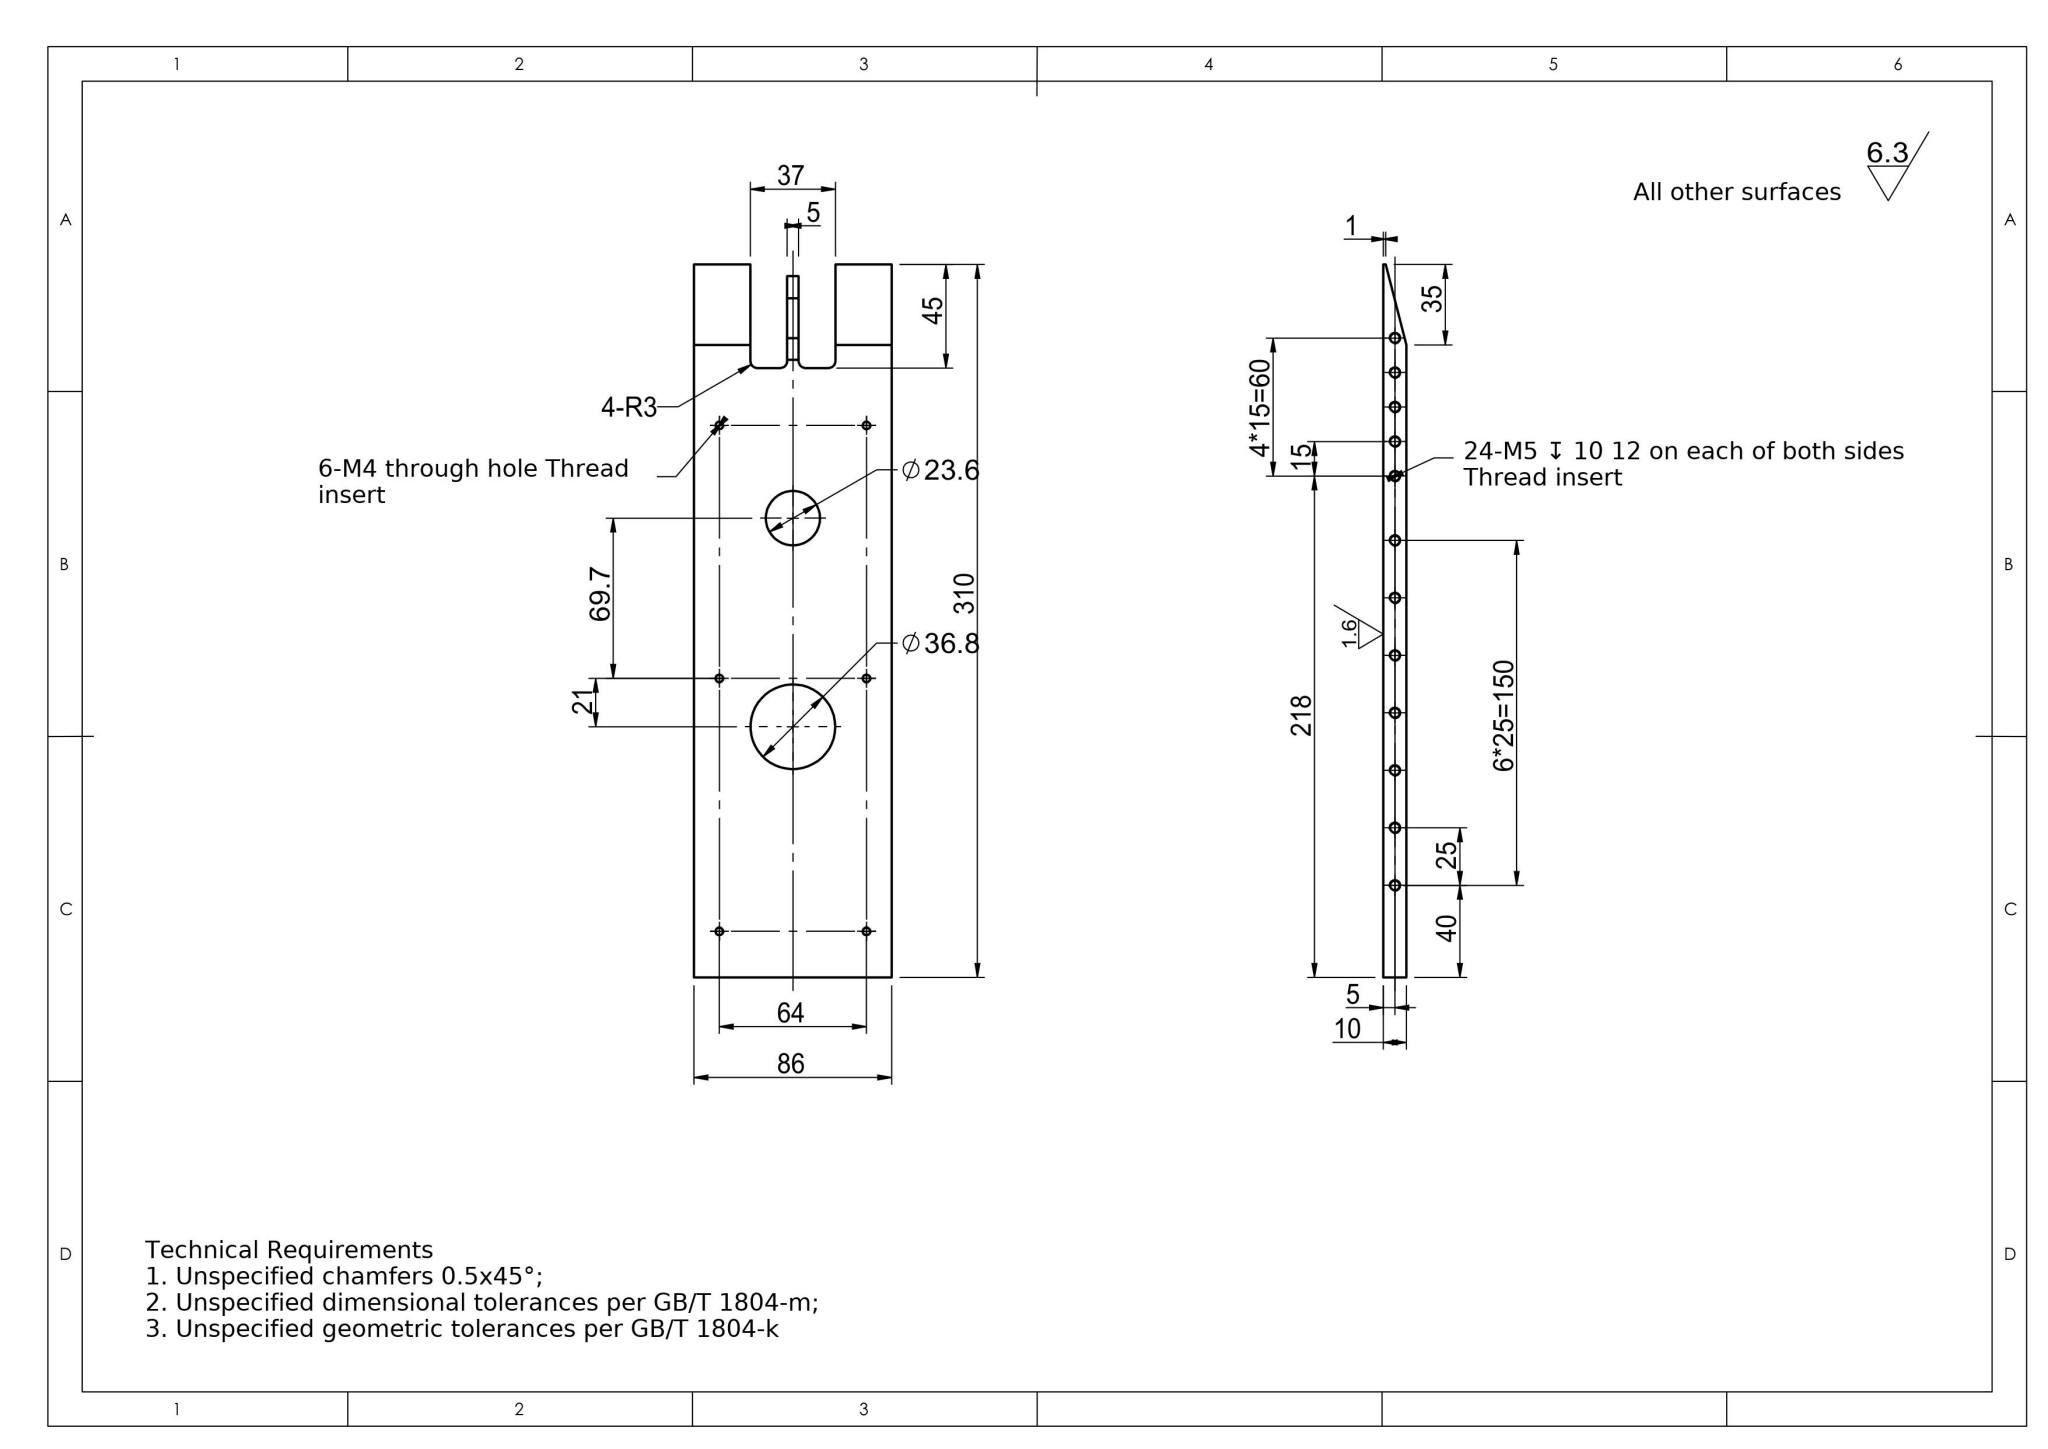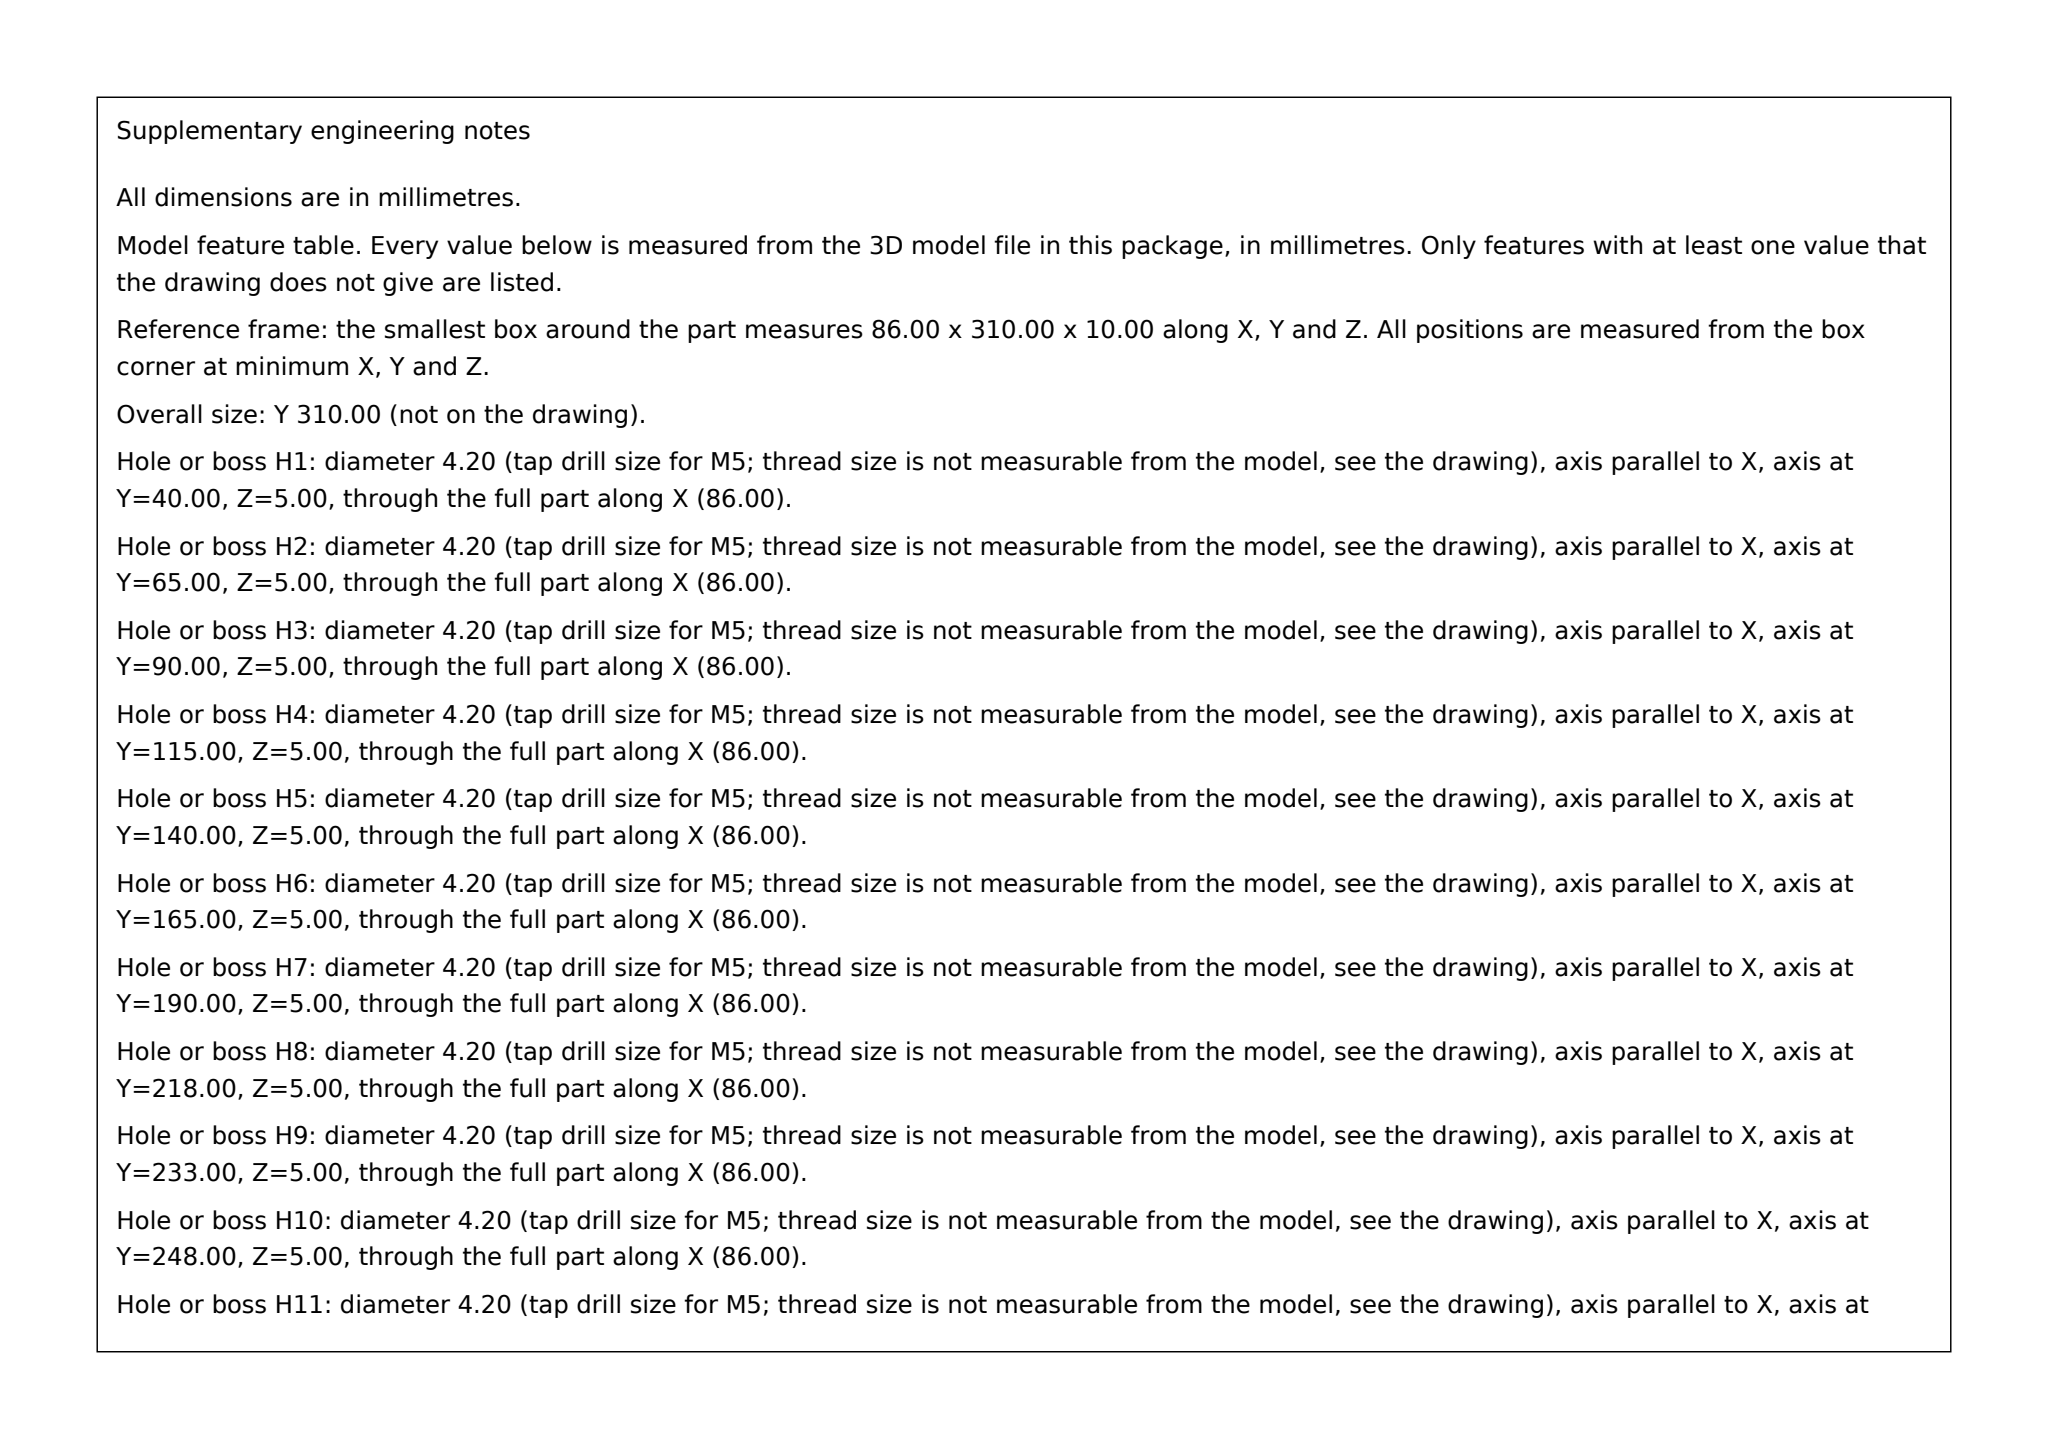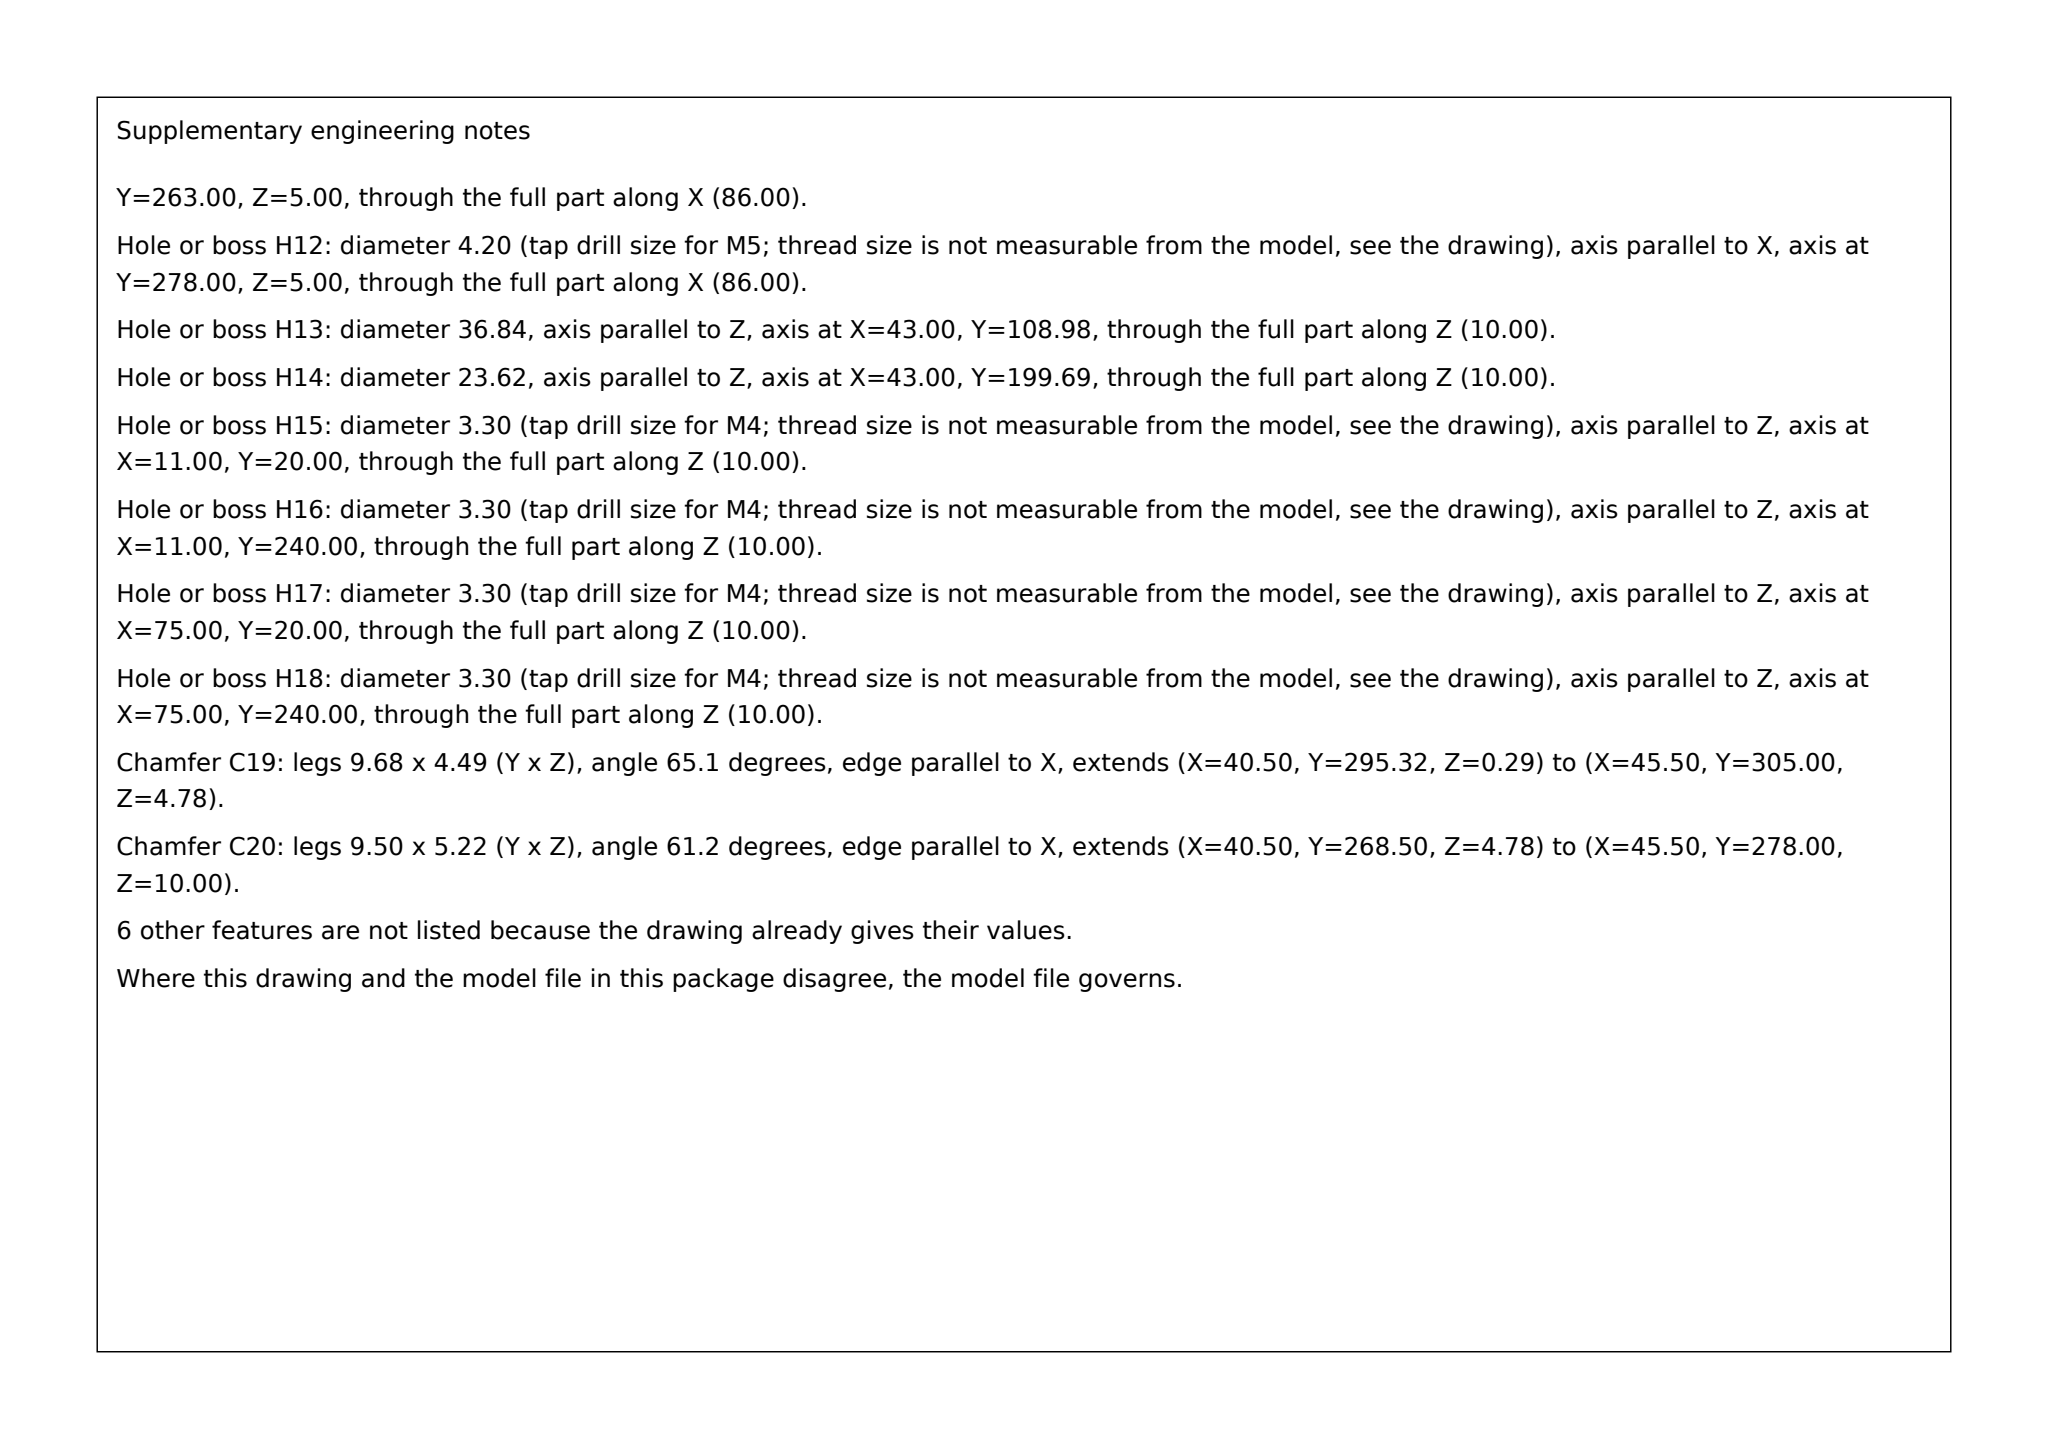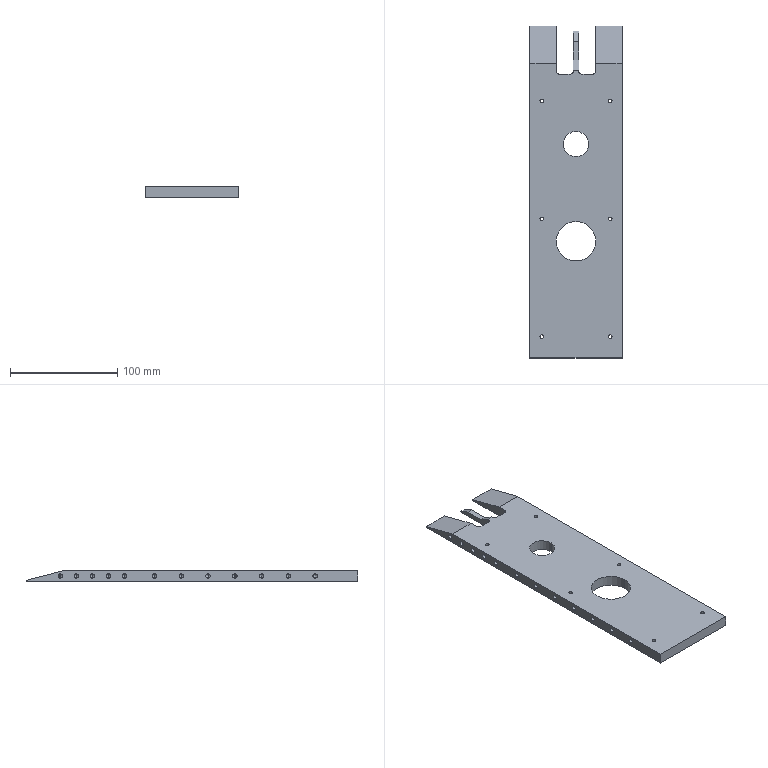Part | SolidWorks | mm | 1 solid | 135 faces | box 86 x 310 x 10 mm | volume 223545 mm3 | cylinder 68 | cone 48 | plane 19 | commonest cylinder face diameters 4.2 x48 3.3 x12 6 x4 23.629 x2 36.85 x2